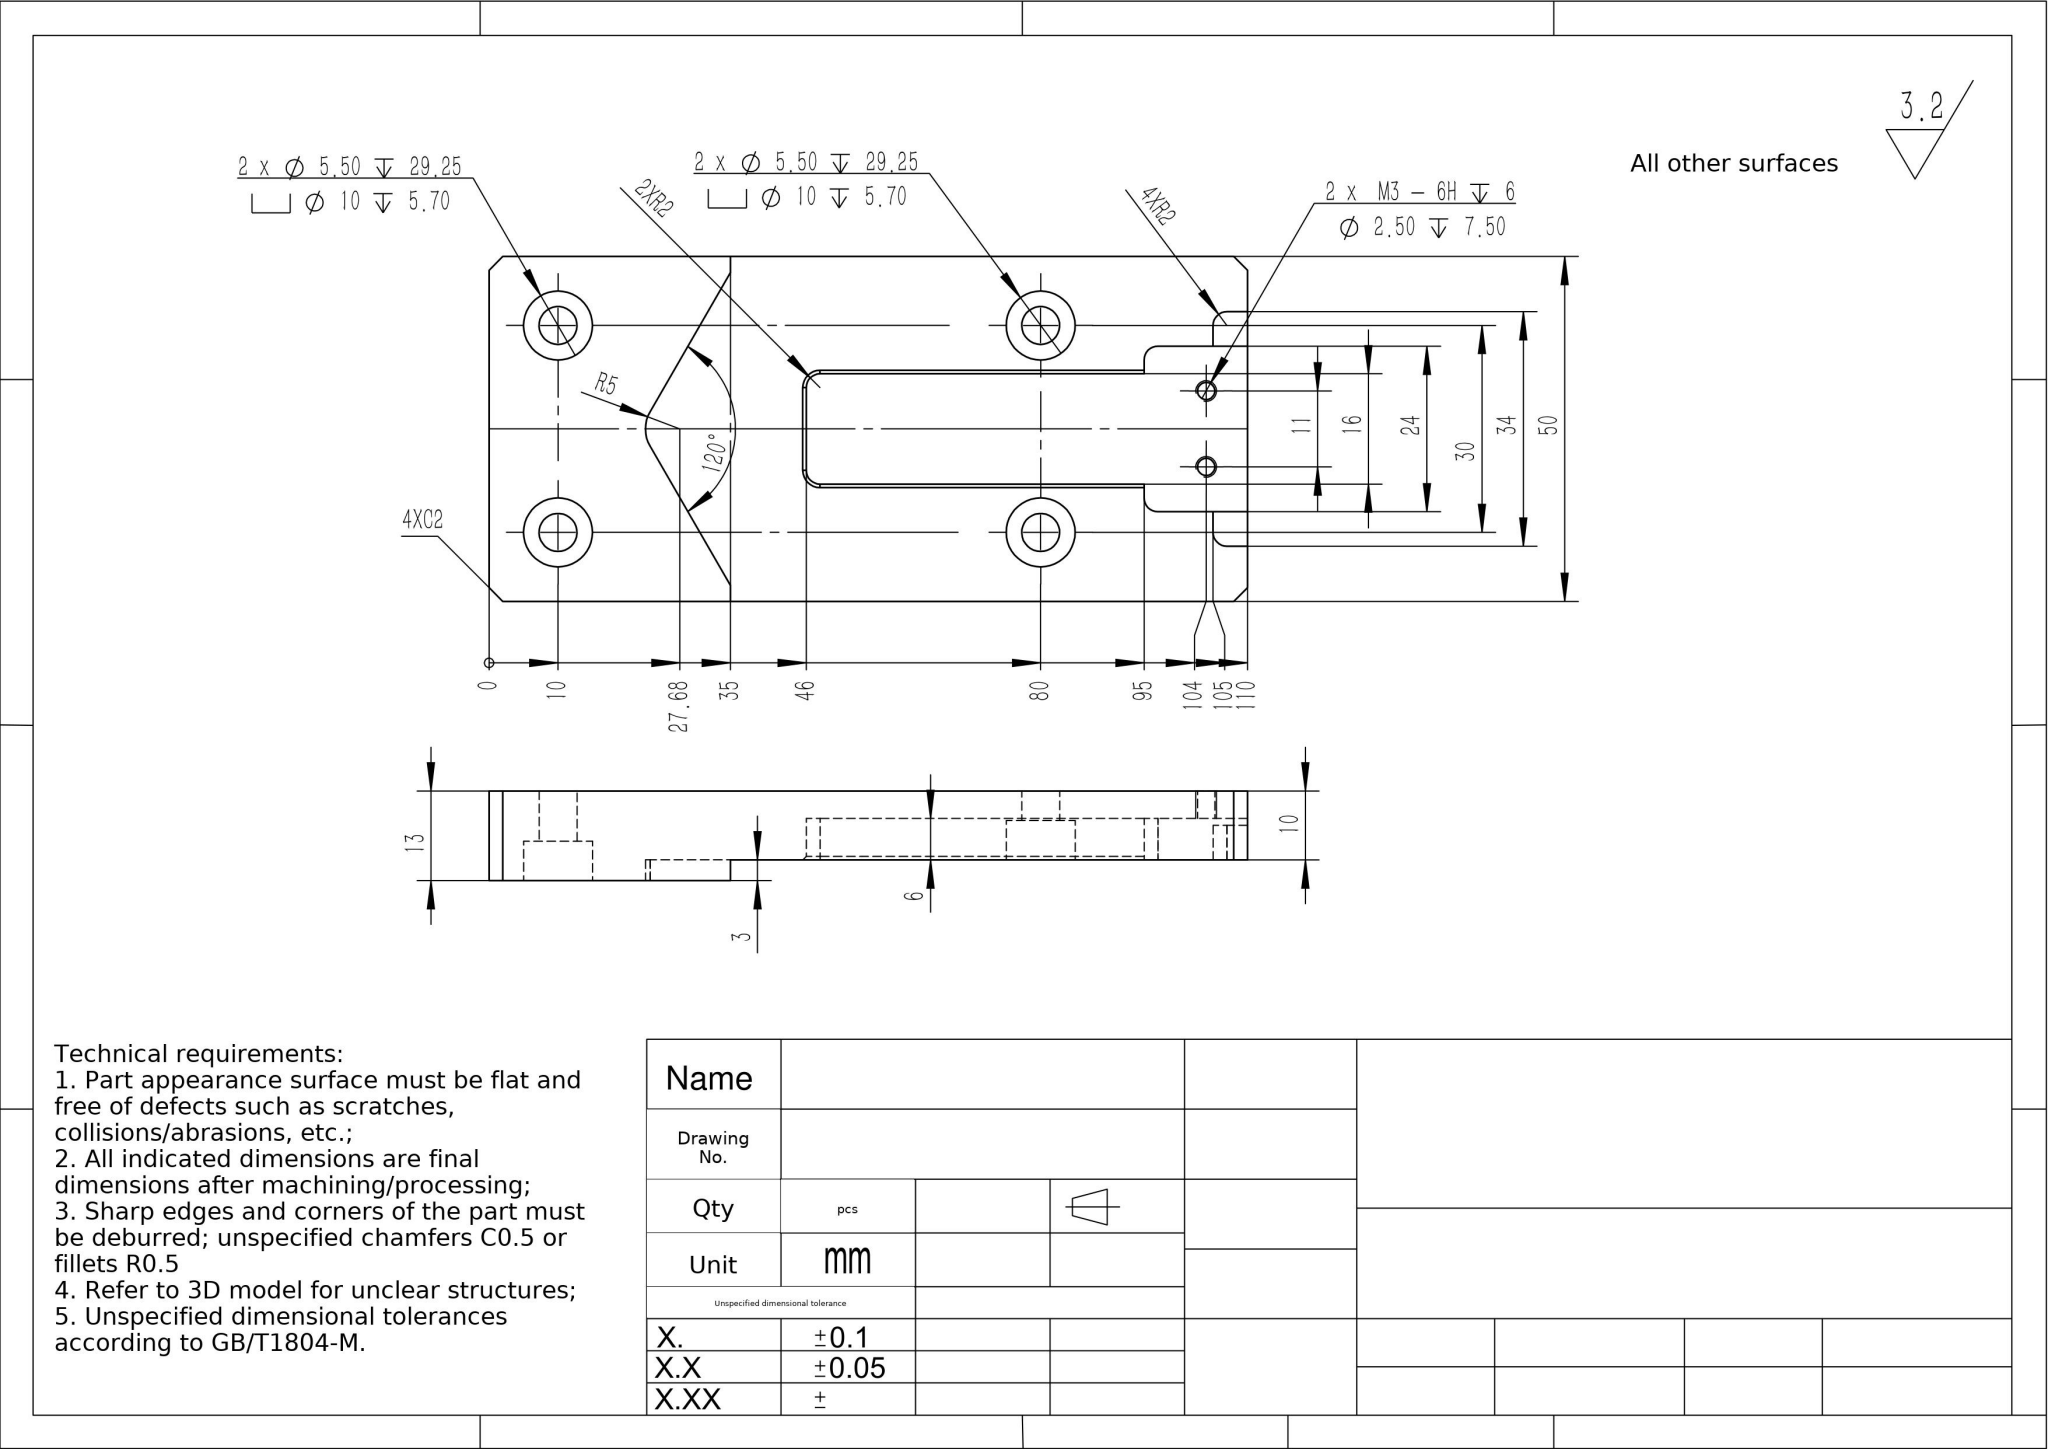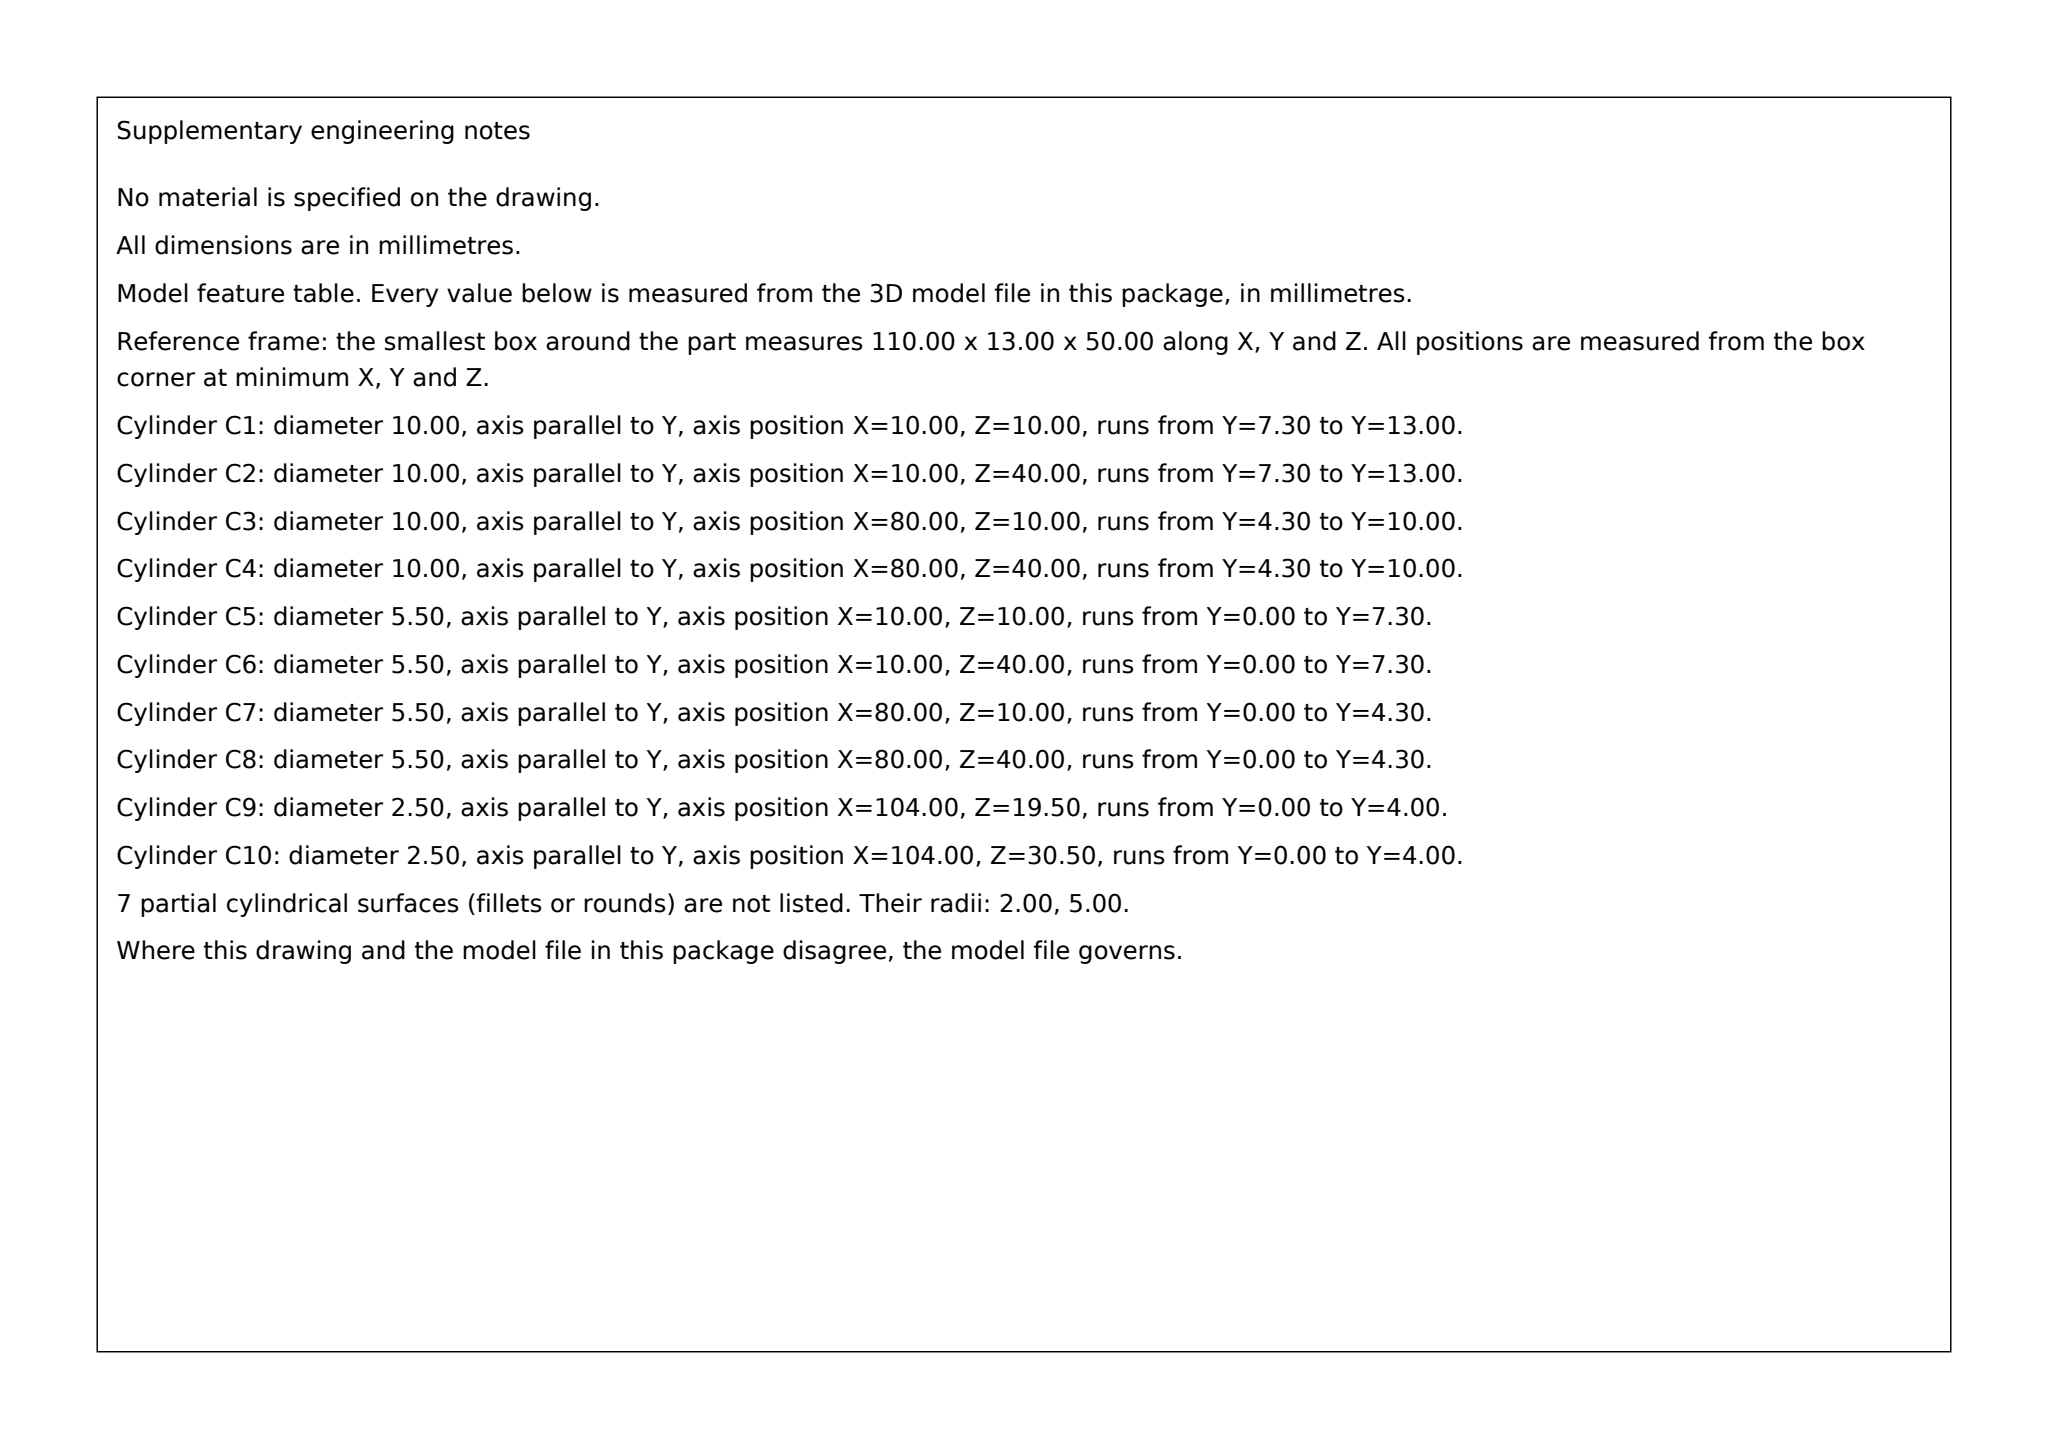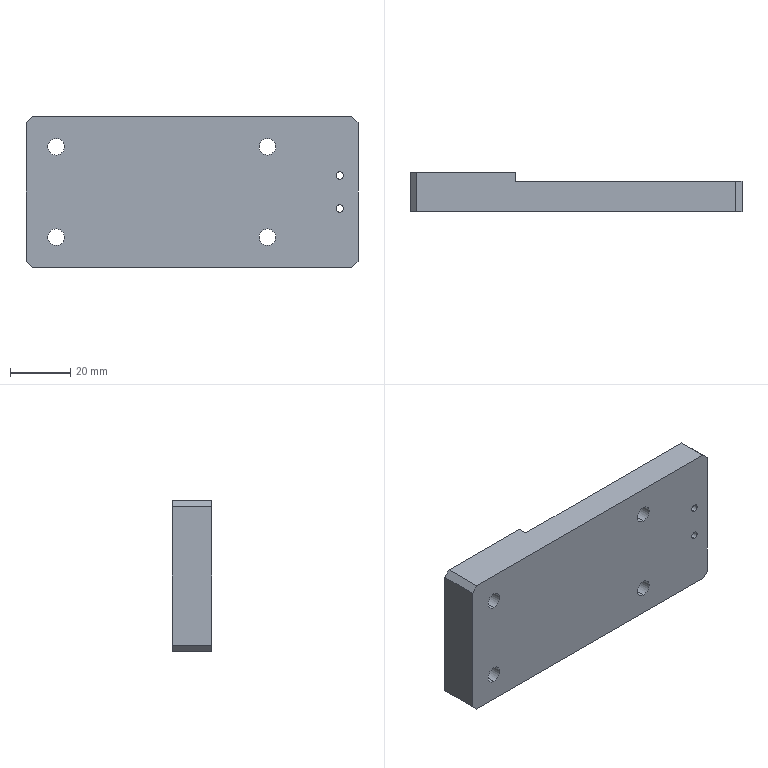Part | SolidWorks | mm | 1 solid | 65 faces | box 110 x 13 x 50 mm | volume 49791 mm3 | plane 36 | cylinder 27 | cone 2 | commonest cylinder face diameters 10 x9 5.5 x8 4 x6 2.5 x4
build123d program:
from build123d import *

# Parameters (mm, degrees)
SKETCH1_W                                           = 110
SKETCH1_H                                           = 50
BOSS_EXTRUDE1_DEPTH                                 = 10
BOSS_EXTRUDE2_DEPTH                                 = 3
HOLE_SIZE_ACCORDING_TO_HEXAGON_SOCKET_H_D           = 5.5
HOLE_SIZE_ACCORDING_TO_HEXAGON_SOCKET_H_DEPTH       = 29.25
HOLE_SIZE_ACCORDING_TO_HEXAGON_SOCKET_H_CBORE_D     = 10
HOLE_SIZE_ACCORDING_TO_HEXAGON_SOCKET_H_CBORE_DEPTH = 5.7
HOLE_SIZE_ACCORDING_TO_HEXAGON_SOCKET_H_TIP         = 1.652
HOLE_SIZE_ACCORDING_TO_HEXAGON_SOCK_2_D             = 5.5
HOLE_SIZE_ACCORDING_TO_HEXAGON_SOCK_2_DEPTH         = 29.25
HOLE_SIZE_ACCORDING_TO_HEXAGON_SOCK_2_CBORE_D       = 10
HOLE_SIZE_ACCORDING_TO_HEXAGON_SOCK_2_CBORE_DEPTH   = 5.7
HOLE_SIZE_ACCORDING_TO_HEXAGON_SOCK_2_TIP           = 1.652
FILLET1_R                                           = 5
CHAMFER1_SIZE                                       = 2
CUT_EXTRUDE1_DEPTH                                  = 6
M3_TAPPED_HOLE1_D                                   = 2.5
M3_TAPPED_HOLE1_DEPTH                               = 7.5
M3_TAPPED_HOLE1_TIP                                 = 0.7511
FILLET2_R                                           = 2
CHAMFER2_SIZE                                       = 0.5
SKETCH11_W                                          = 10
SKETCH11_H                                          = 34
CUT_EXTRUDE2_DEPTH                                  = 5
FILLET3_R                                           = 2


with BuildPart() as part:
    # Sketch1 → Boss-Extrude1 (new body)
    with BuildSketch(Plane(origin=(0, 0, 0), x_dir=(1, 0, 0), z_dir=(0, 1, 0))):
        Rectangle(SKETCH1_W, SKETCH1_H)
    extrude(amount=BOSS_EXTRUDE1_DEPTH)

    # Sketch2 → Boss-Extrude2 (add)
    with BuildSketch(Plane(origin=(0, 10, 0), x_dir=(1, 0, 0), z_dir=(0, 1, 0))):
        Polygon((-33.094, 0), (-20, 22.679), (-20, 25), (-55, 25), (-55, -25), (-20, -25), (-20, -22.679), align=None)
    extrude(amount=BOSS_EXTRUDE2_DEPTH)

    # Hole Size_ According to_Hexagon Socket H
    with Locations(Plane(origin=(25, 10, 15), x_dir=(0, 0, 1), z_dir=(0, 1, 0))):
        with Locations((0, 0), (-30, 0)):
            CounterBoreHole(HOLE_SIZE_ACCORDING_TO_HEXAGON_SOCKET_H_D / 2, HOLE_SIZE_ACCORDING_TO_HEXAGON_SOCKET_H_CBORE_D / 2, HOLE_SIZE_ACCORDING_TO_HEXAGON_SOCKET_H_CBORE_DEPTH, depth=HOLE_SIZE_ACCORDING_TO_HEXAGON_SOCKET_H_DEPTH)
            with Locations((0, 0, -(HOLE_SIZE_ACCORDING_TO_HEXAGON_SOCKET_H_DEPTH + HOLE_SIZE_ACCORDING_TO_HEXAGON_SOCKET_H_TIP / 2))):  # 118° drill point
                Cone(0, HOLE_SIZE_ACCORDING_TO_HEXAGON_SOCKET_H_D / 2, HOLE_SIZE_ACCORDING_TO_HEXAGON_SOCKET_H_TIP, mode=Mode.SUBTRACT)

    # Hole Size_ According to_Hexagon Sock 2
    with Locations(Plane(origin=(-45, 13, -15), x_dir=(0, 0, 1), z_dir=(0, 1, 0))):
        with Locations((0, 0), (30, 0)):
            CounterBoreHole(HOLE_SIZE_ACCORDING_TO_HEXAGON_SOCK_2_D / 2, HOLE_SIZE_ACCORDING_TO_HEXAGON_SOCK_2_CBORE_D / 2, HOLE_SIZE_ACCORDING_TO_HEXAGON_SOCK_2_CBORE_DEPTH, depth=HOLE_SIZE_ACCORDING_TO_HEXAGON_SOCK_2_DEPTH)
            with Locations((0, 0, -(HOLE_SIZE_ACCORDING_TO_HEXAGON_SOCK_2_DEPTH + HOLE_SIZE_ACCORDING_TO_HEXAGON_SOCK_2_TIP / 2))):  # 118° drill point
                Cone(0, HOLE_SIZE_ACCORDING_TO_HEXAGON_SOCK_2_D / 2, HOLE_SIZE_ACCORDING_TO_HEXAGON_SOCK_2_TIP, mode=Mode.SUBTRACT)

    # Fillet1
    fillet1_edges = [part.edges().sort_by_distance(p)[0] for p in [
        (-33.094, 11.5, 0),
    ]]
    fillet(fillet1_edges, radius=FILLET1_R)

    # Chamfer1
    chamfer1_edges = [part.edges().sort_by_distance(p)[0] for p in [
        (55, 5, 25),
        (-55, 6.5, 25),
        (-55, 6.5, -25),
        (55, 5, -25),
    ]]
    chamfer(chamfer1_edges, length=CHAMFER1_SIZE)

    # Sketch8 → Cut-Extrude1 (cut)
    with BuildSketch(Plane(origin=(0, 10, 0), x_dir=(1, 0, 0), z_dir=(0, 1, 0))):
        with BuildLine():
            Line((-7, 8), (40, 8))
            Line((40, 8), (40, 12))
            Line((40, 12), (55, 12))
            Line((55, 12), (55, -12))
            Line((55, -12), (40, -12))
            Line((40, -12), (40, -8))
            Line((40, -8), (-7, -8))
            ThreePointArc((-7, -8), (-8.414, -7.414), (-9, -6))
            Line((-9, -6), (-9, 6))
            ThreePointArc((-9, 6), (-8.414, 7.414), (-7, 8))
        make_face()
    extrude(amount=-CUT_EXTRUDE1_DEPTH, mode=Mode.SUBTRACT)

    # M3 Tapped Hole1
    with Locations(Plane(origin=(49, 4, 5.5), x_dir=(0, 0, 1), z_dir=(0, 1, 0))):
        with Locations((0, 0), (-11, 0)):
            Hole(M3_TAPPED_HOLE1_D / 2, depth=M3_TAPPED_HOLE1_DEPTH)
            with Locations((0, 0, -(M3_TAPPED_HOLE1_DEPTH + M3_TAPPED_HOLE1_TIP / 2))):  # 118° drill point
                Cone(0, M3_TAPPED_HOLE1_D / 2, M3_TAPPED_HOLE1_TIP, mode=Mode.SUBTRACT)

    # Fillet2
    fillet2_edges = [part.edges().sort_by_distance(p)[0] for p in [
        (40, 7, -12),
        (40, 7, 12),
    ]]
    fillet(fillet2_edges, radius=FILLET2_R)

    # Chamfer2
    chamfer2_edges = [part.edges().sort_by_distance(p)[0] for p in [
        (16.5, 10, -8),
        (-8.414, 10, -7.414),
        (-9, 10, 0),
        (-8.414, 10, 7.414),
        (16.5, 10, 8),
    ]]
    chamfer(chamfer2_edges, length=CHAMFER2_SIZE)

    # Sketch11 → Cut-Extrude2 (cut)
    with BuildSketch(Plane(origin=(0, 10, 0), x_dir=(1, 0, 0), z_dir=(0, 1, 0))):
        with Locations((55, 0)):
            Rectangle(SKETCH11_W, SKETCH11_H)
    extrude(amount=-CUT_EXTRUDE2_DEPTH, mode=Mode.SUBTRACT)

    # Fillet3
    fillet3_edges = [part.edges().sort_by_distance(p)[0] for p in [
        (50, 7.5, -17),
        (50, 7.5, 17),
    ]]
    fillet(fillet3_edges, radius=FILLET3_R)


solid = part.part